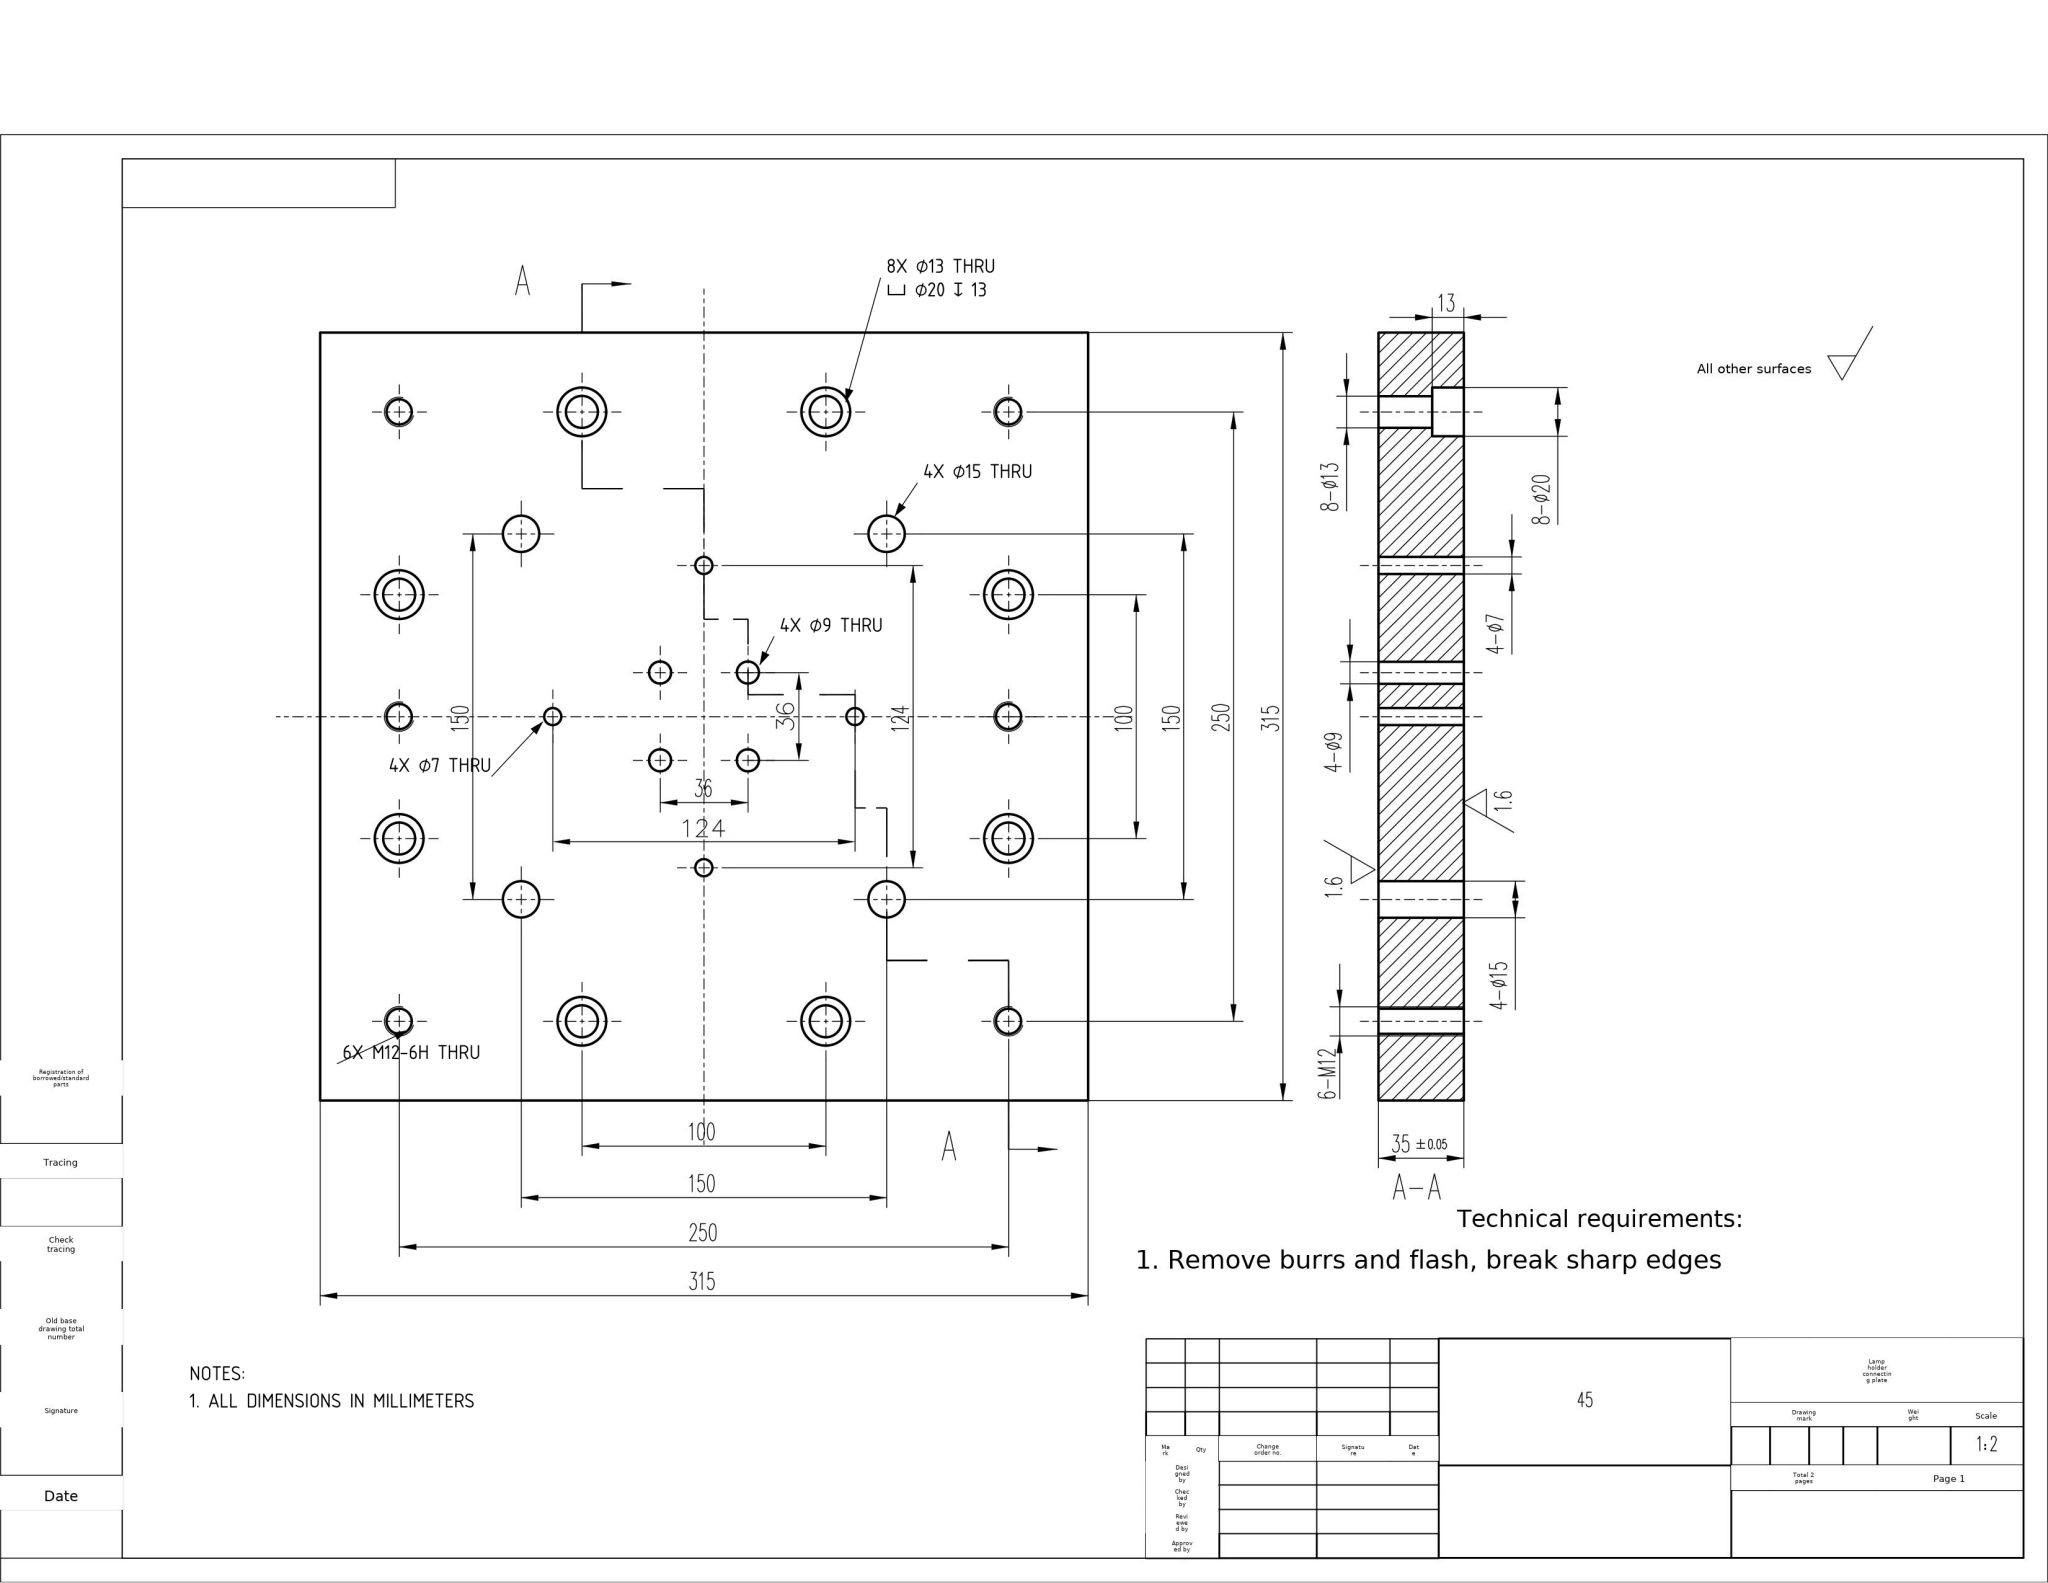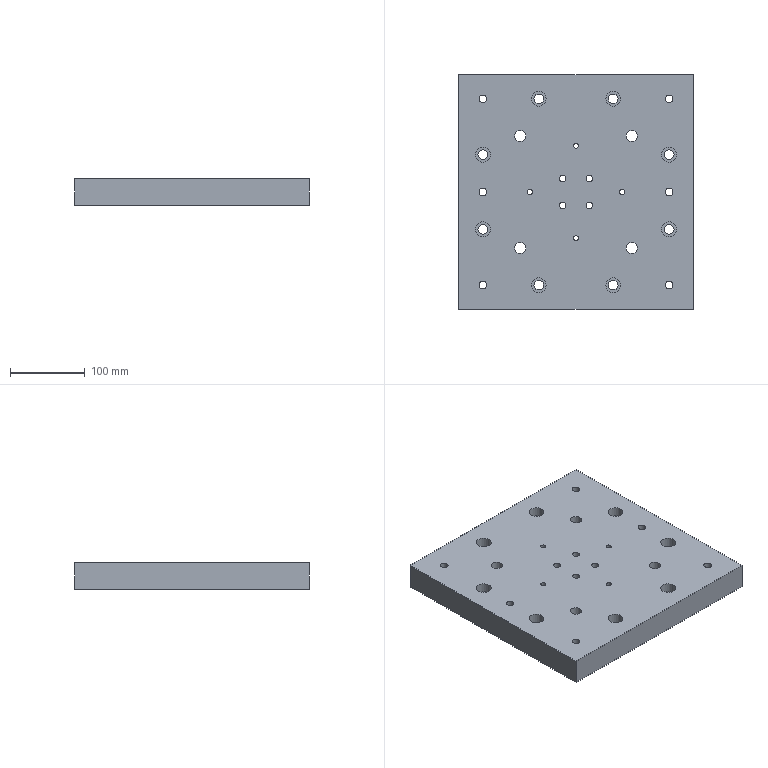Part | NX | mm | 1 solid | 48 faces | box 315 x 315 x 35 mm | volume 3360309 mm3 | cylinder 34 | plane 14 | commonest cylinder face diameters 13 x8 20 x8 10.3 x6 15 x4 7 x4 9 x4